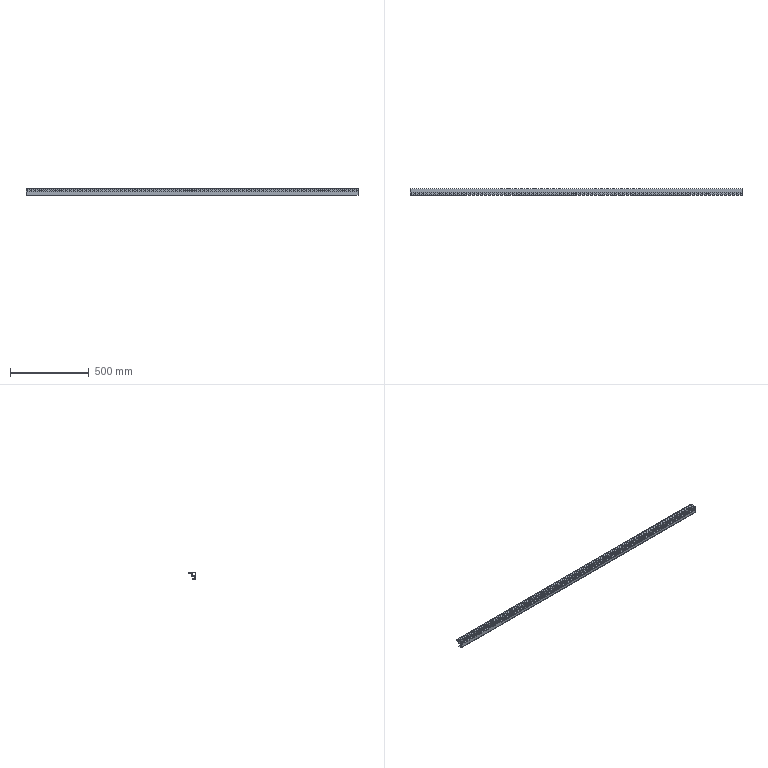Component | SolidWorks | CabinetFrameWeldmentDrawingPG50-01-00-1_RightColumnPG50-01-102-1 | 4 solids | 1122 faces | volume 606928 mm3 | plane 708 | cylinder 414 | commonest cylinder face diameters 4.1 x340 6.532 x18 6.5 x8 1 x8 8.8 x6 3.999 x6 15 x6 6 x6 | material AISI 1045 Steel, cold drawn